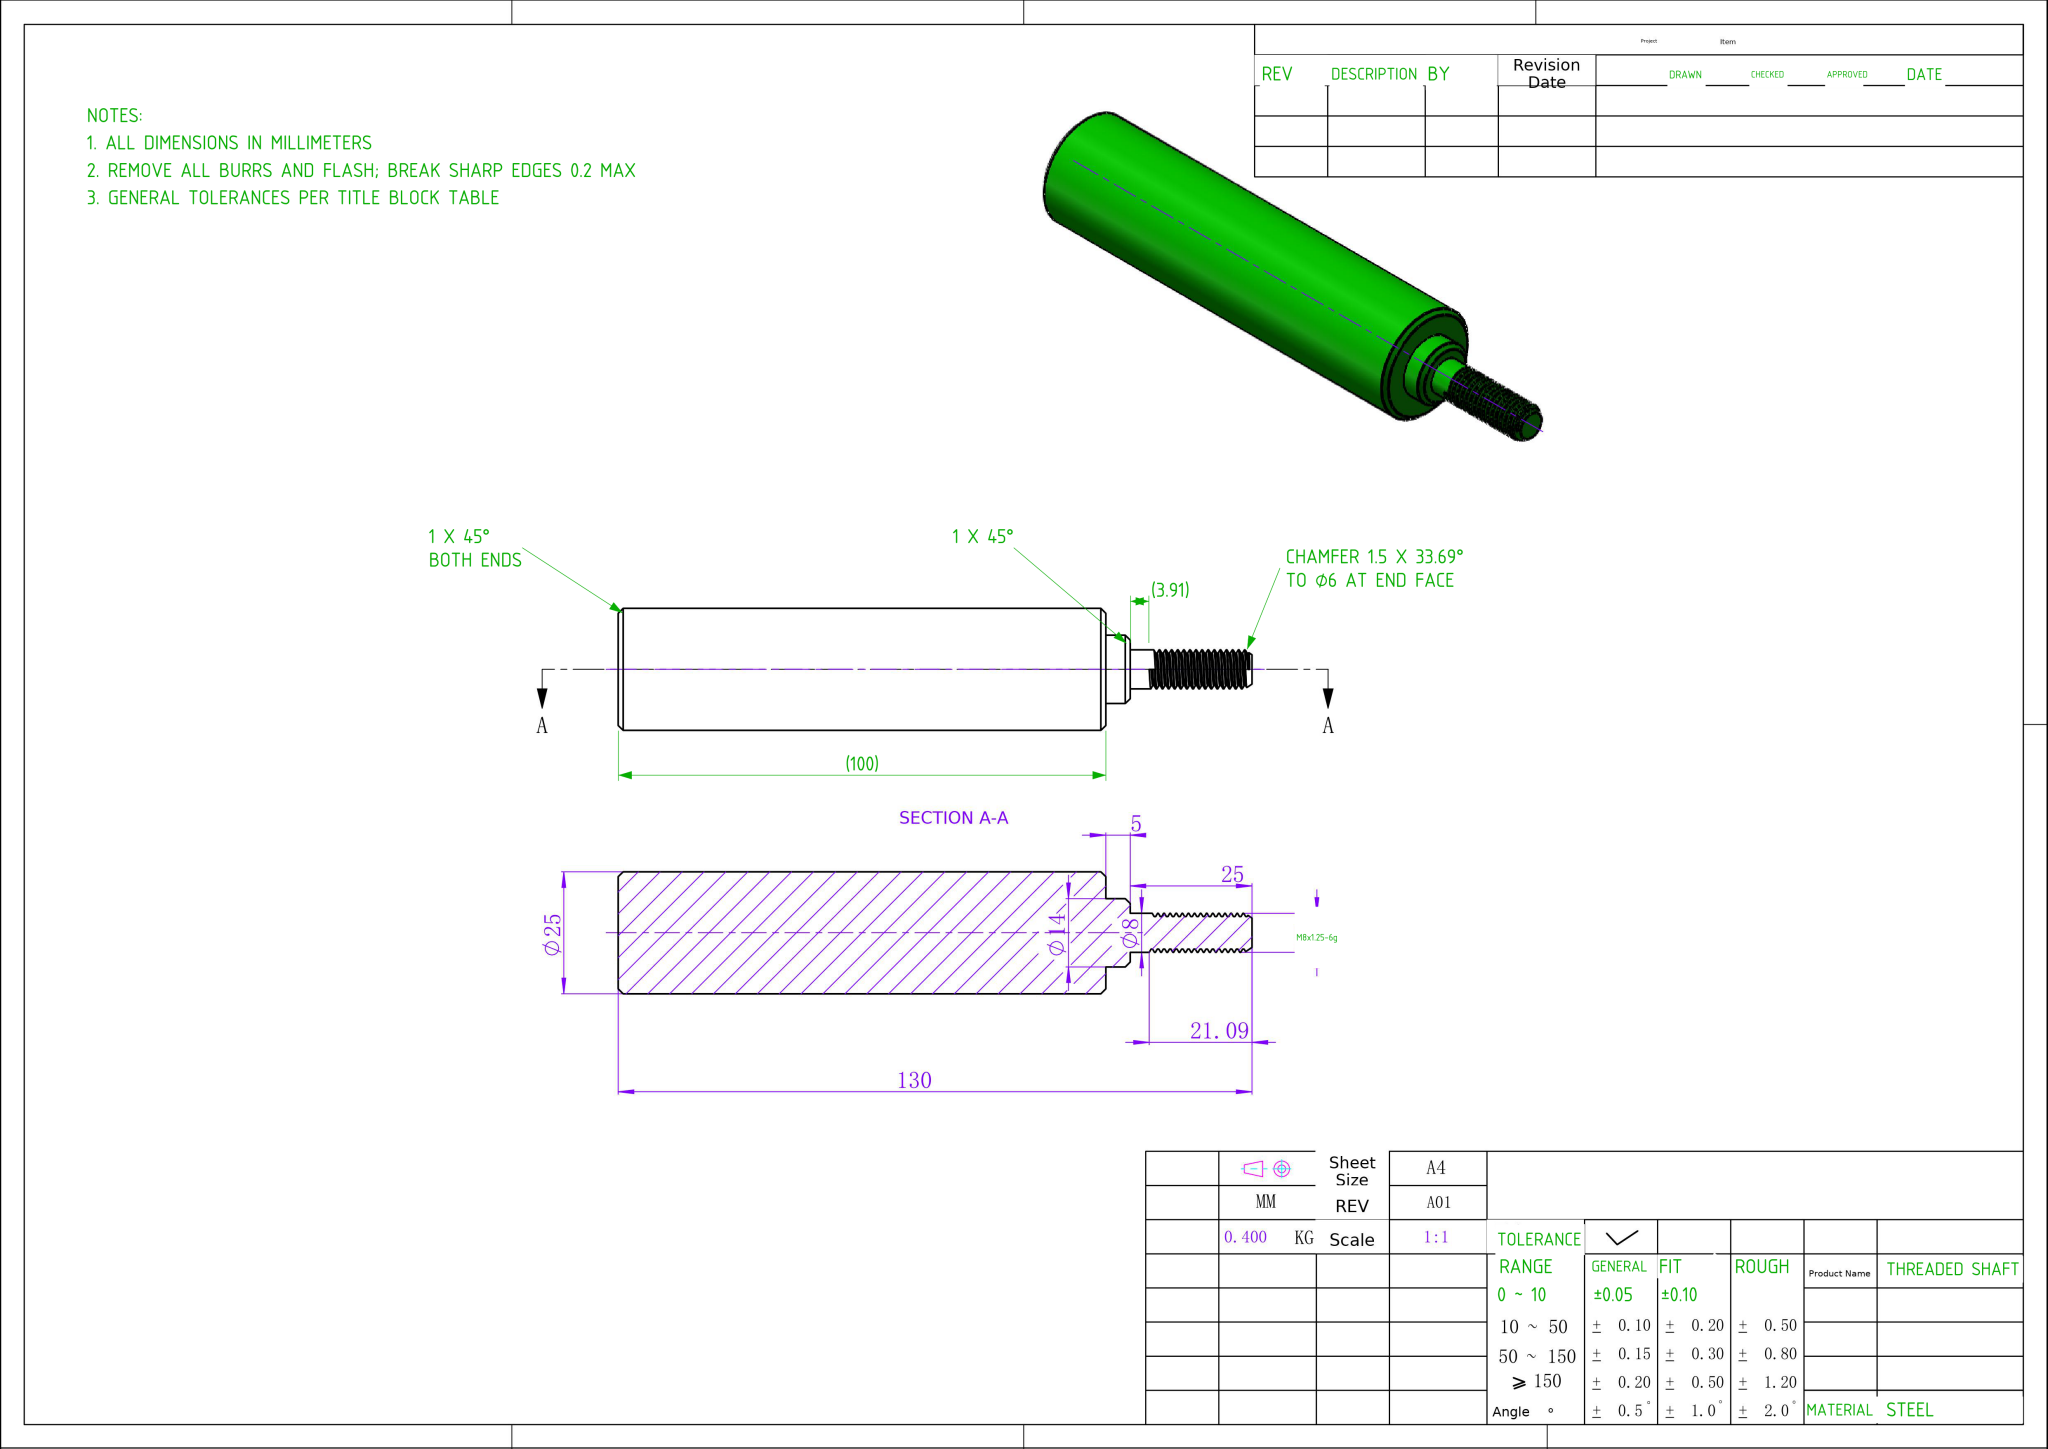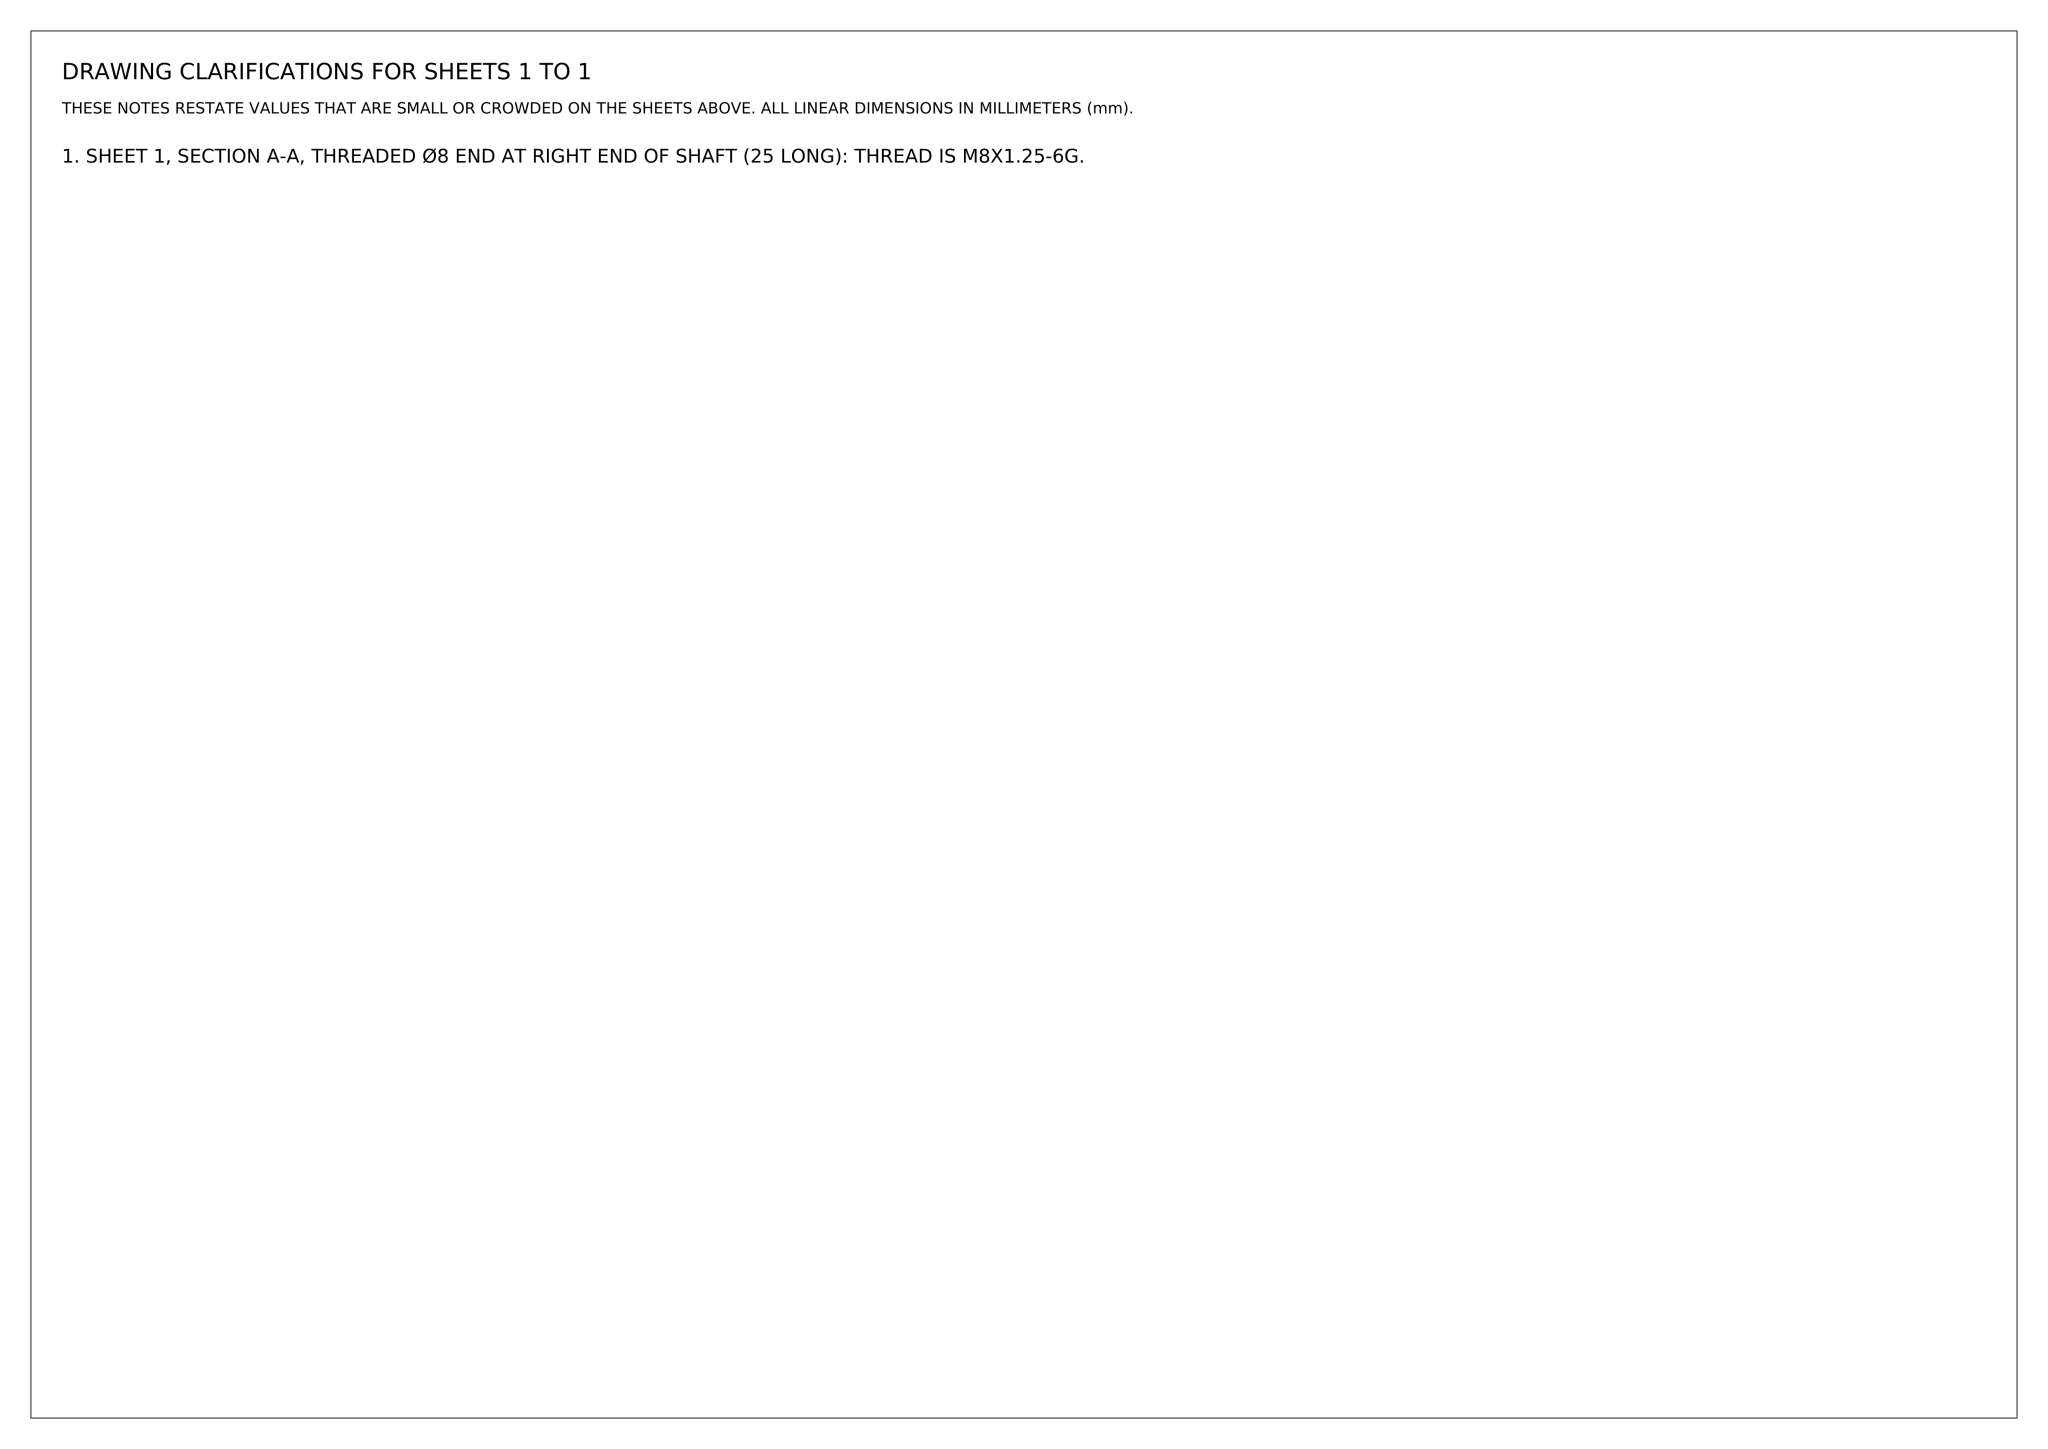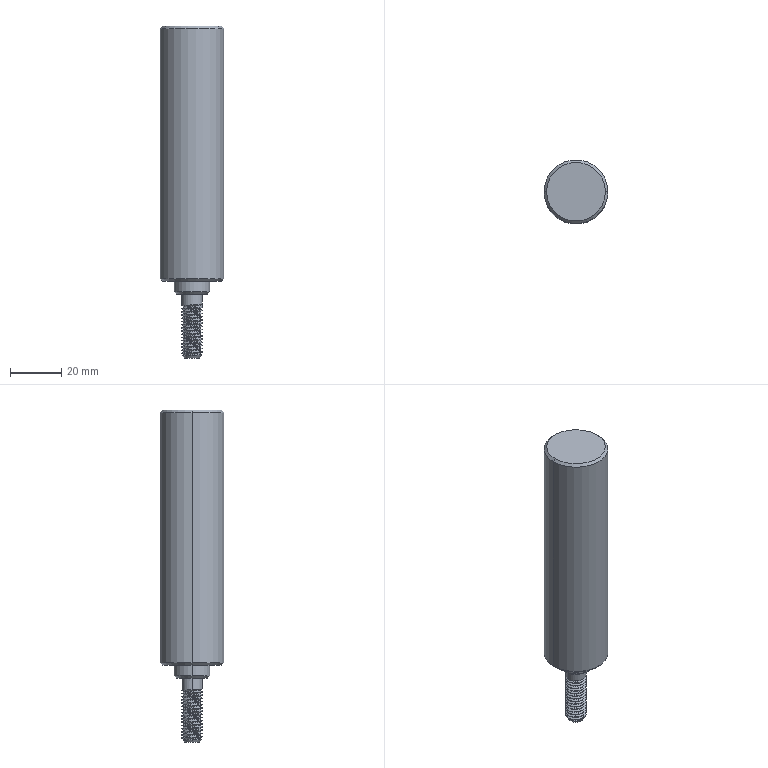Part | NX | mm | 1 solid | 54 faces | box 25 x 25 x 130 mm | volume 50826 mm3 | cylinder 36 | cone 9 | plane 6 | spline 3 | commonest cylinder face diameters 8 x32 14 x2 25 x2